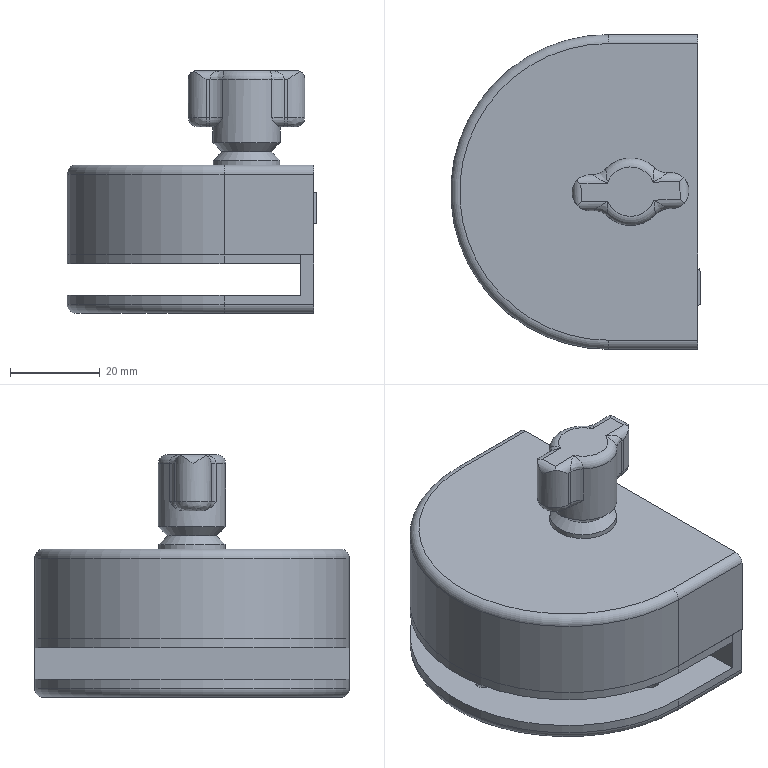Assembly | NX | mm | 5 component files | 5 solids | 146 faces | box 55.64 x 70 x 54 mm | volume 50480 mm3 | plane 75 | cylinder 41 | cone 16 | torus 8 | spline 6 | commonest cylinder face diameters 4 x16 3.5 x7 8 x6 15 x3 70 x3 46 x1 59 x1 14.8 x1
Bill of materials:
unnamed part 1 | 1 |  | Wing-knob-shaped solid: a central cylindrical hub with two opposed flat-topped lobes (wings), rounded/filleted edges, a chamfered lower hub end, and a slender square-section stem sticking out from the bottom.
unnamed part 2 | 1 |  | Thin flat D-shaped plate (a semicircle merged with a rectangle) with two small upright tabs along the straight edge, each tab having one round through-hole.
unnamed part 3 | 1 |  | D-shaped base plate, thicker than unnamed part 2, with a raised wall along the straight edge, two upright tabs with round holes at the ends of that wall, and three small through-holes spaced around the curved part of the plate.
unnamed part 4 | 1 |  | D-shaped housing or cover-like body with a flat top, a rounded top edge and a flat straight-side wall. The top has one large central round hole. The flat wall has two rectangular openings and two small round holes near its lower corners.
unnamed part 5 | 1 |  | Open C-shaped ring (a ring with a gap) joined by a tapered arm/web to a central cylindrical boss. The boss has a chamfered top end with a small square recess and extends above the ring. A lower layer/lobe projects below the ring under the boss and web.
Mates:
1. fix | lock_body_end_cover 1 component
2. concentric | lock_body 1 edge | lock_body_end_cover 1 edge
3. concentric | lock_body_base_cover 1 edge | lock_body_end_cover 1 edge
4. touch align | fixed 1 face | lock_body_end_cover 1 face
5. touch align | fixed 1 face | lock_body_end_cover 1 face
6. touch align | wrench 1 face | lock_body 1 face
7. touch align | wrench 1 face | lock_body 1 face
8. touch align | wrench 1 face | lock_body 1 face